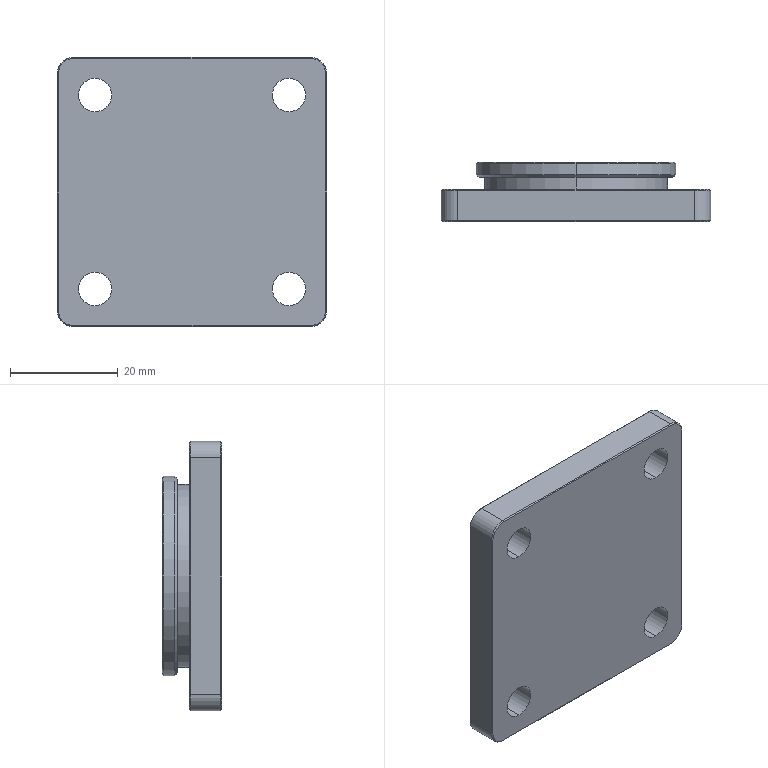CAM job | Mastercam | mm | 4 operations | part box 50 x 11 x 50
1. Contour (Ramp) | 9 - 10 平铣刀
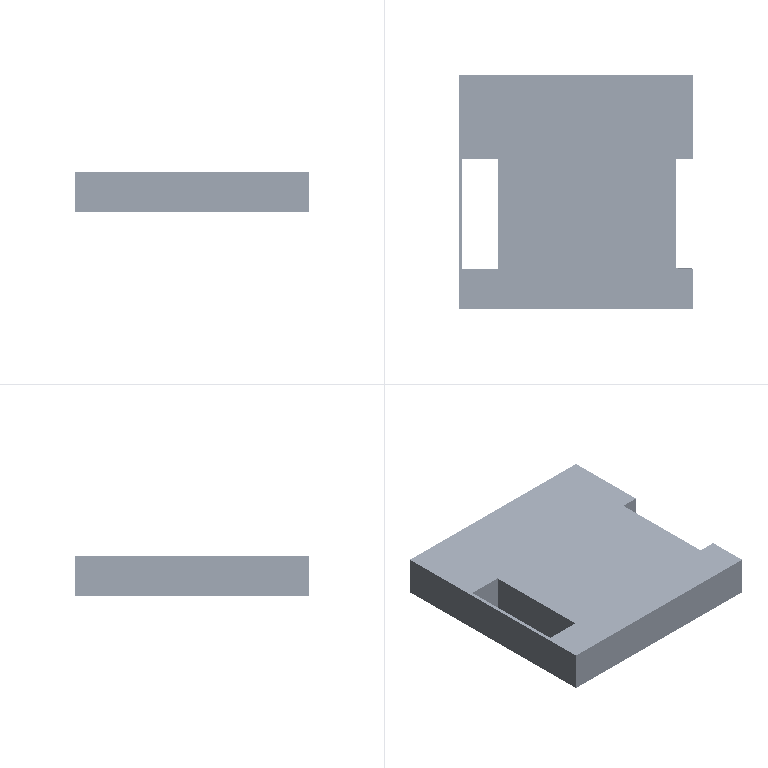2. Contour (2D) | 10 - 10 平铣刀
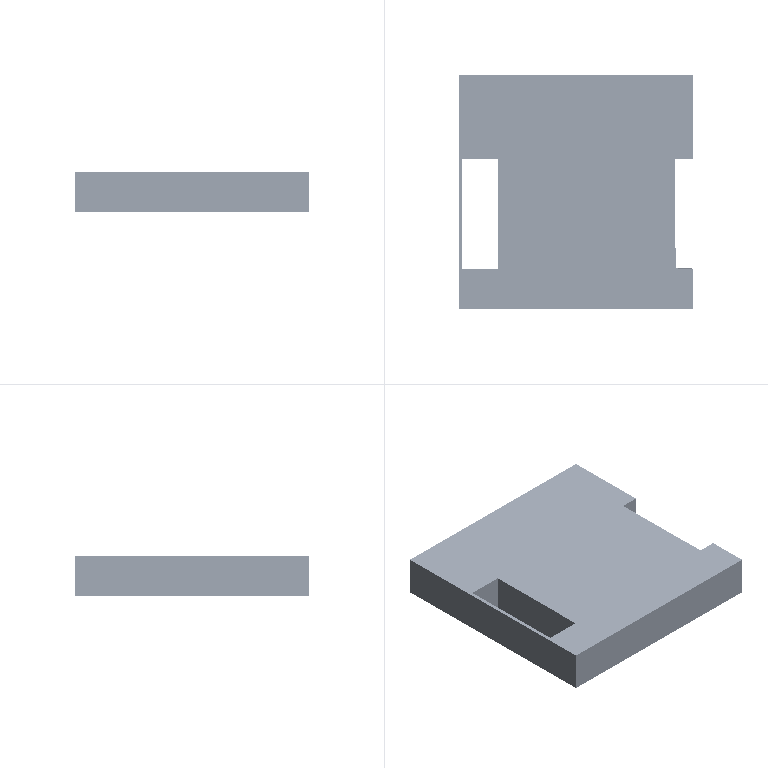3. Drill/Counterbore | 5 - 4 倒角刀
4. Contour (2D chamfer) | 5 - 4 倒角刀